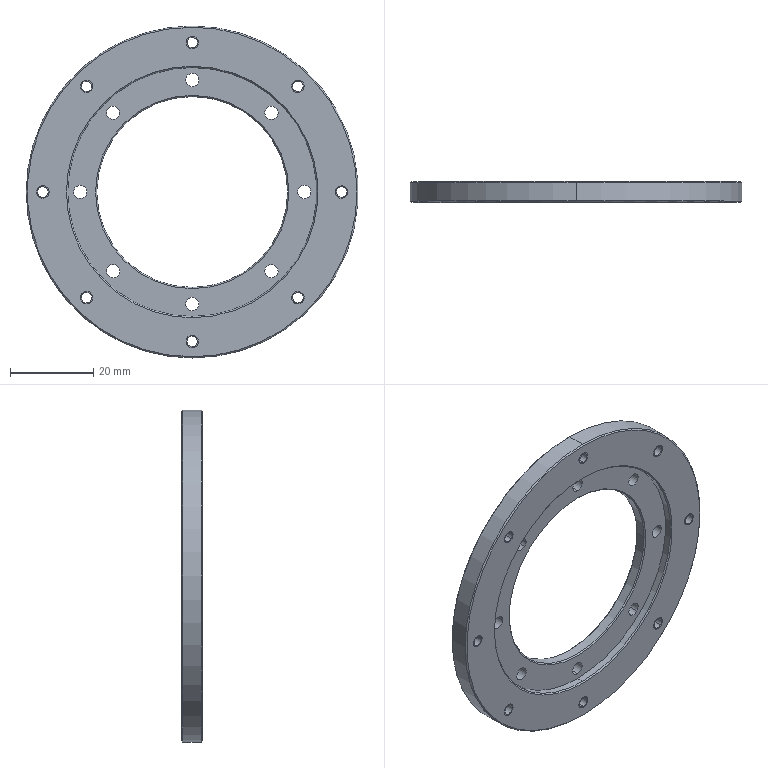CAM job | Mastercam | mm | 1 operations | part box 80 x 5 x 80
1. Drill/Counterbore | 5 - 4 倒角刀